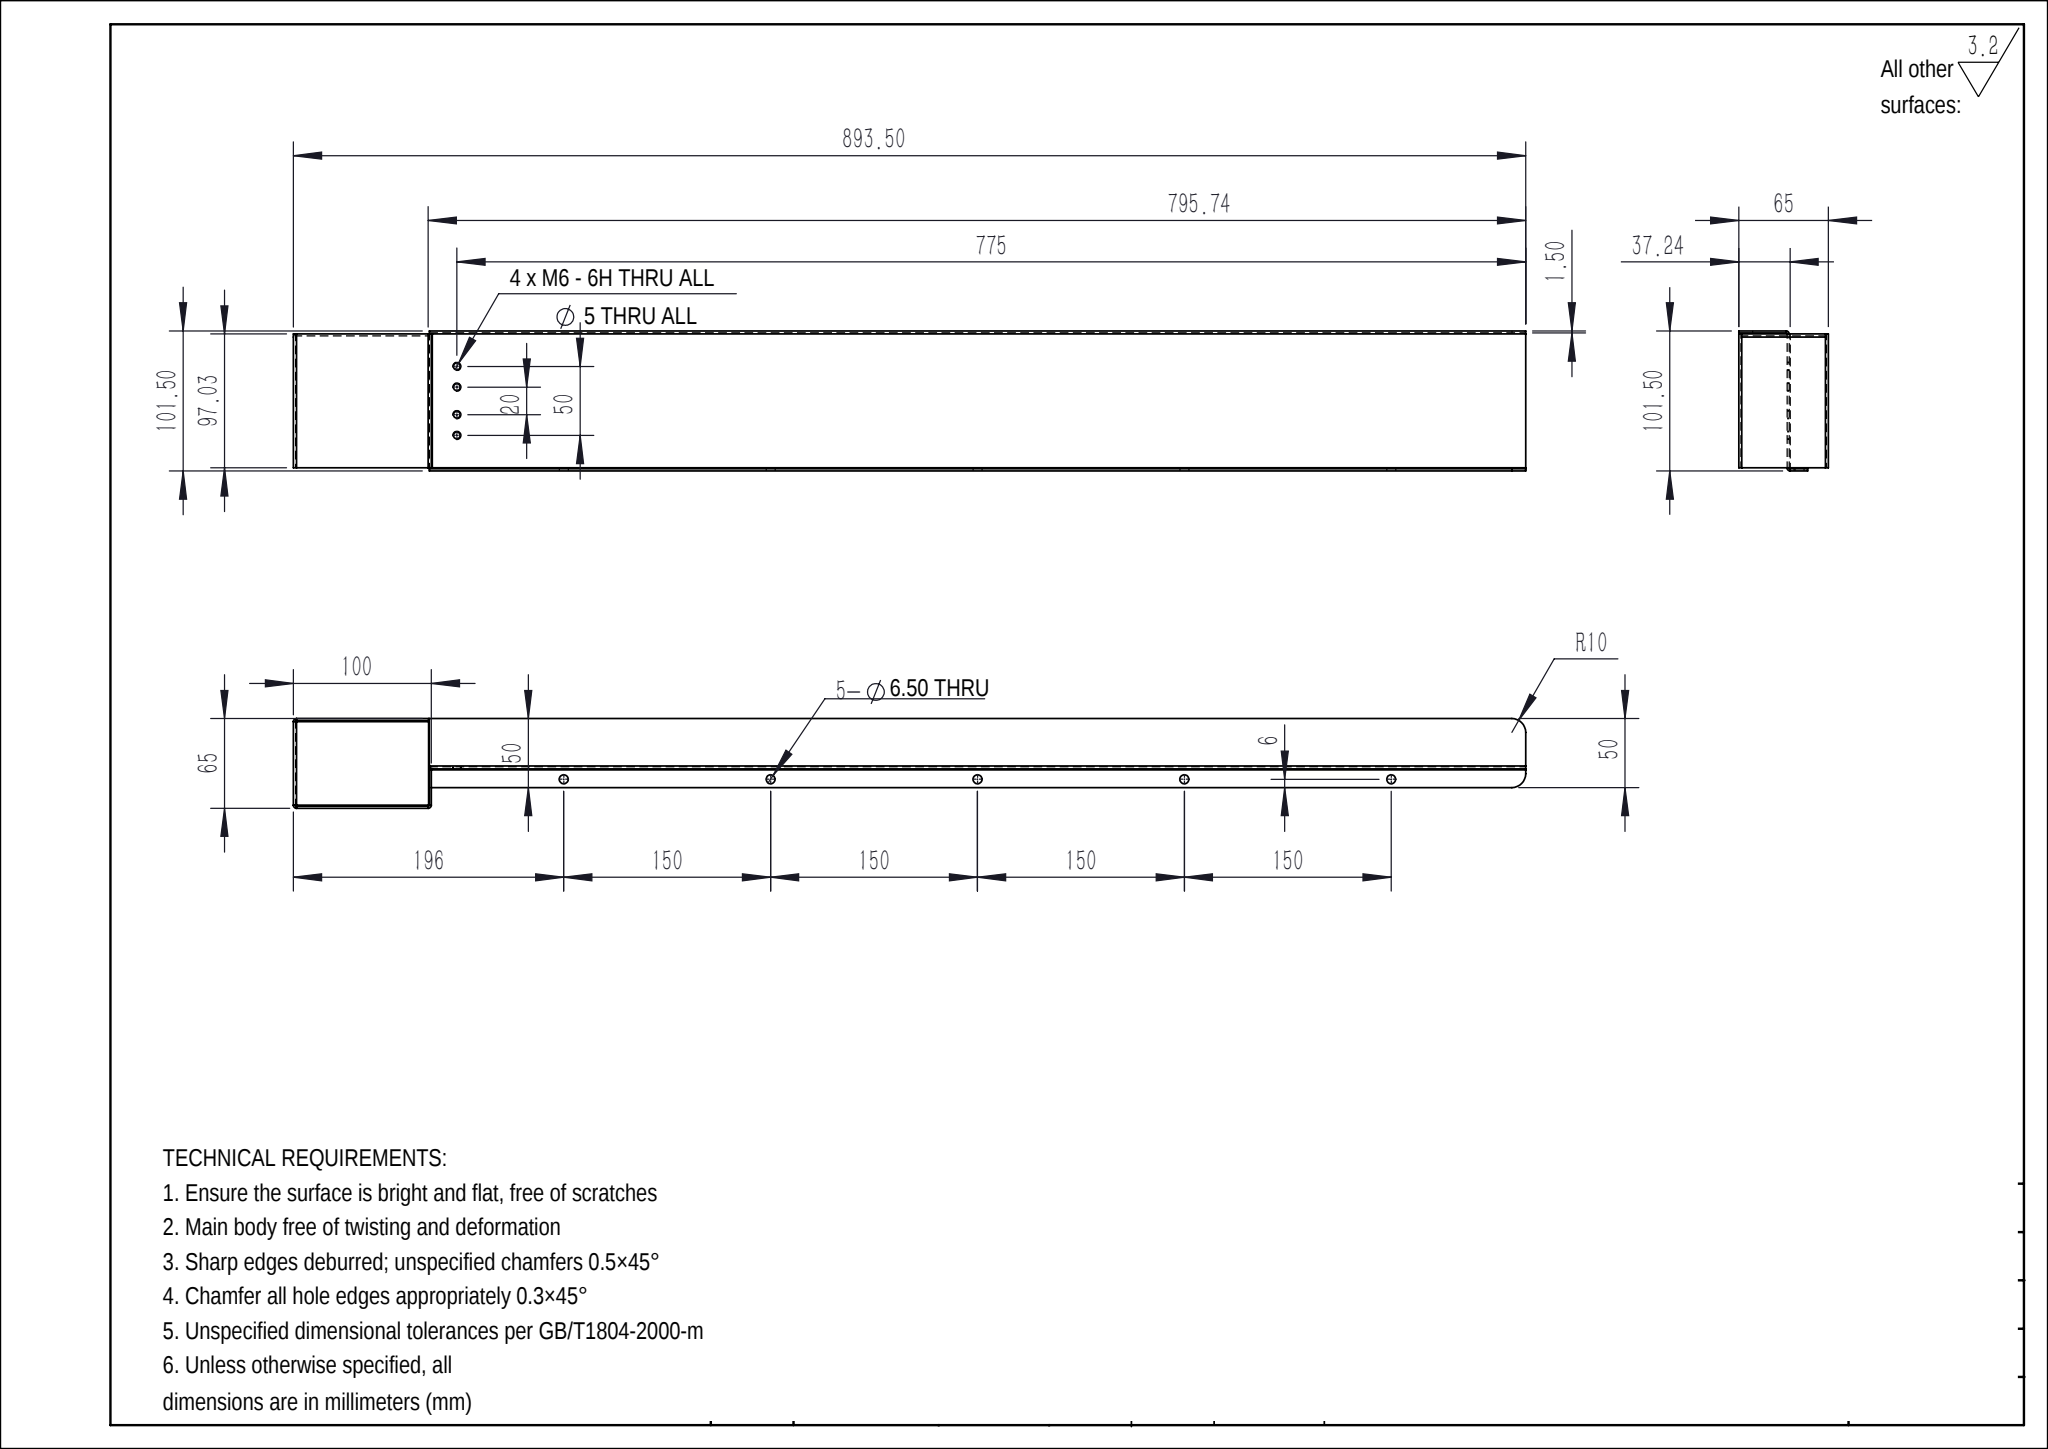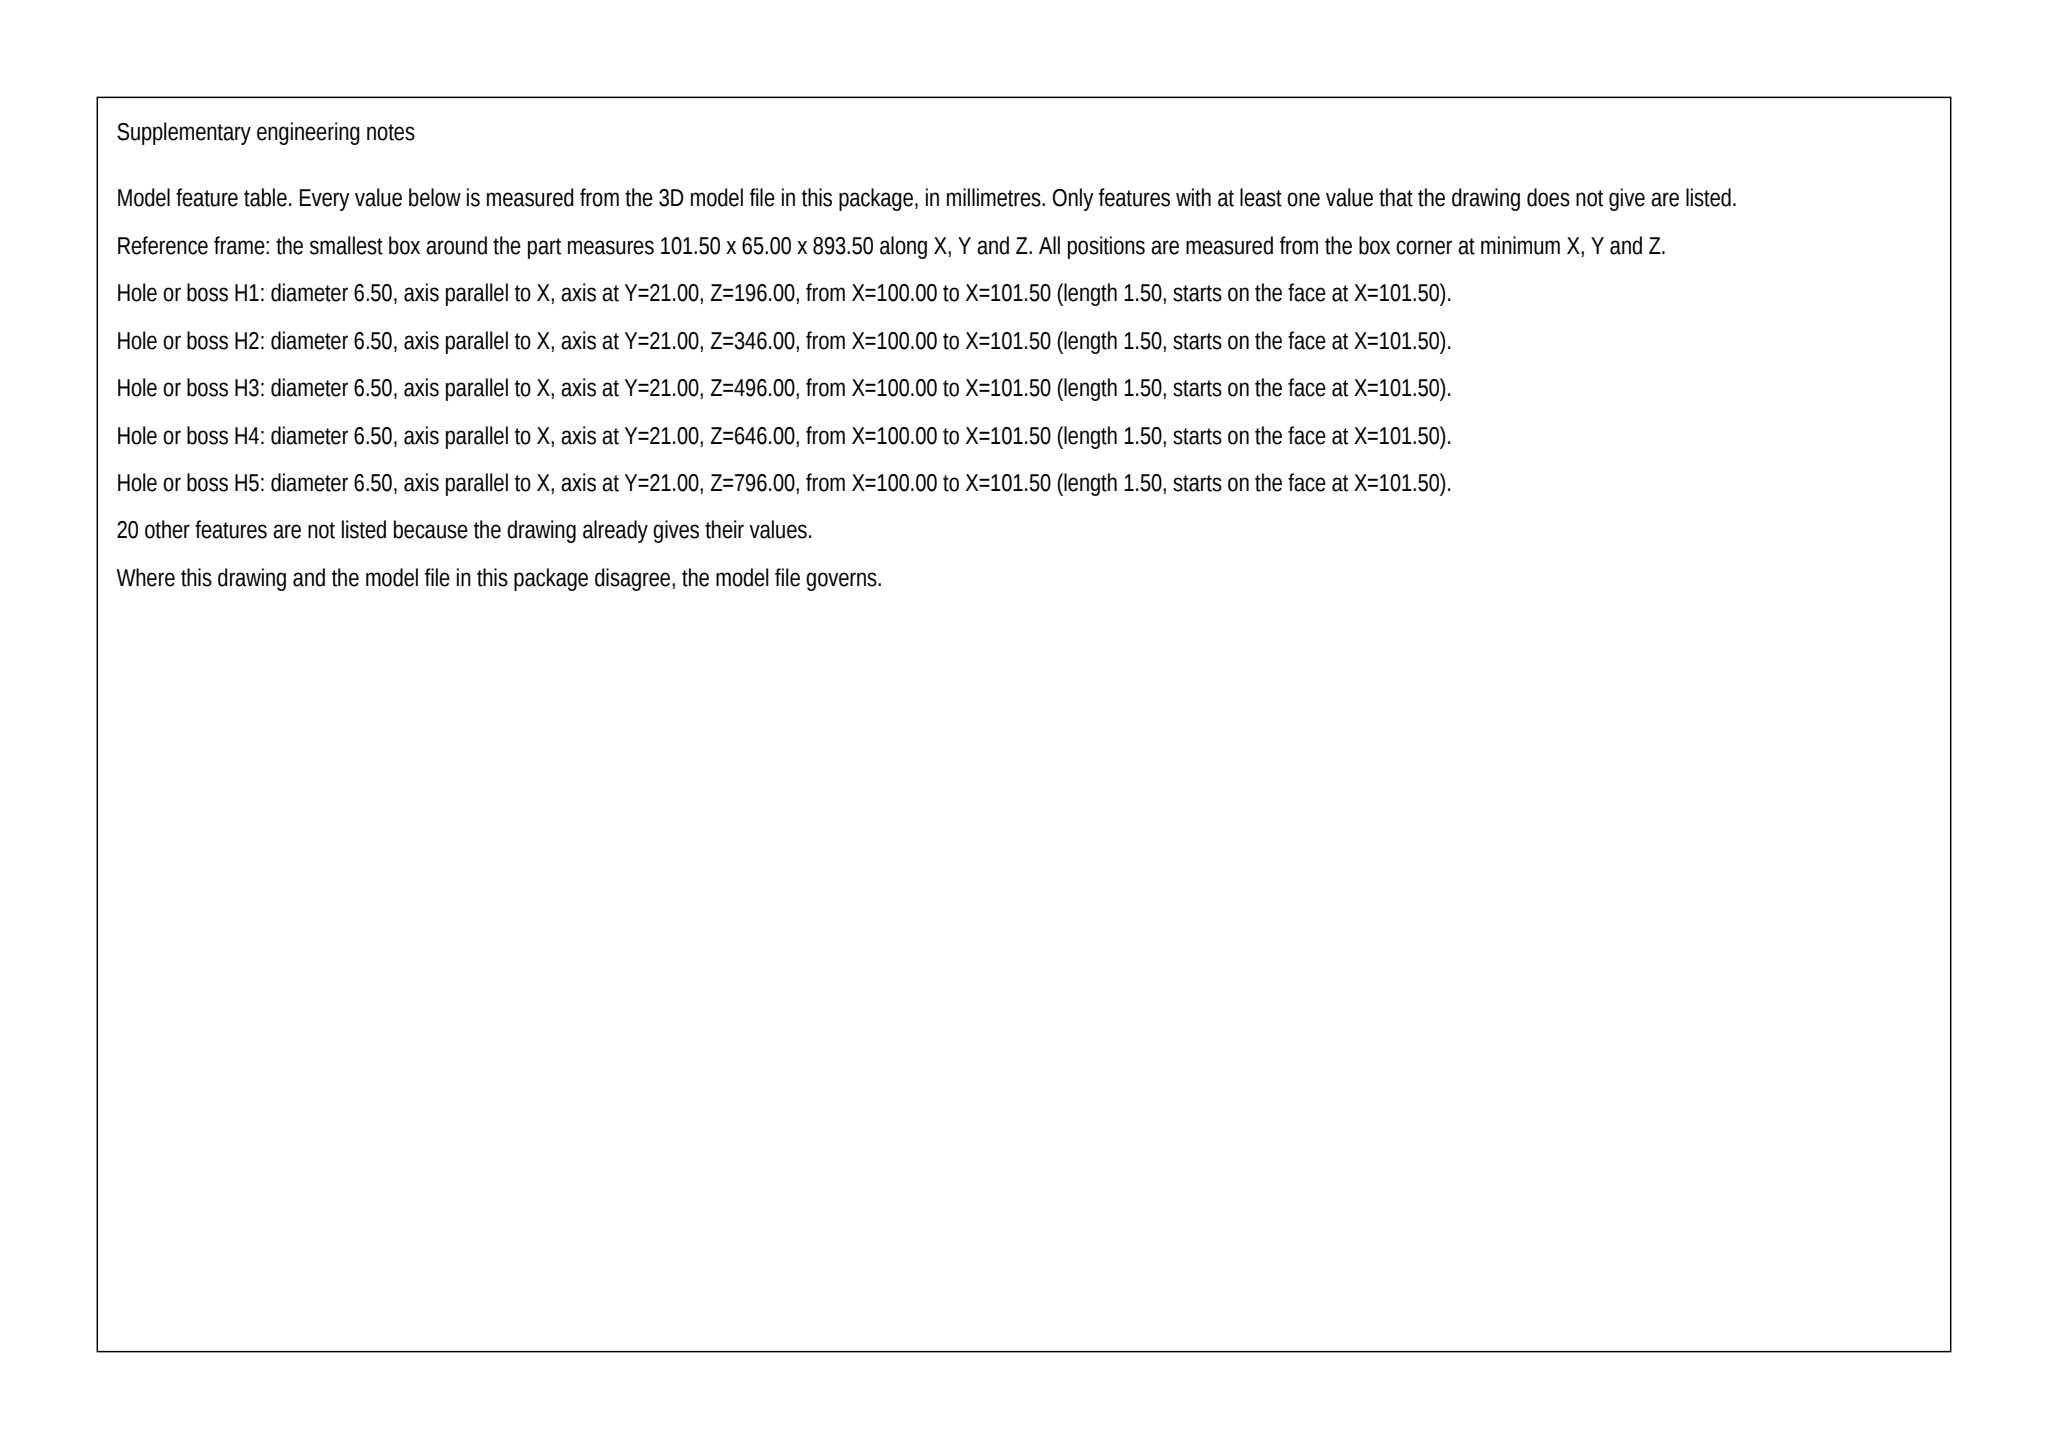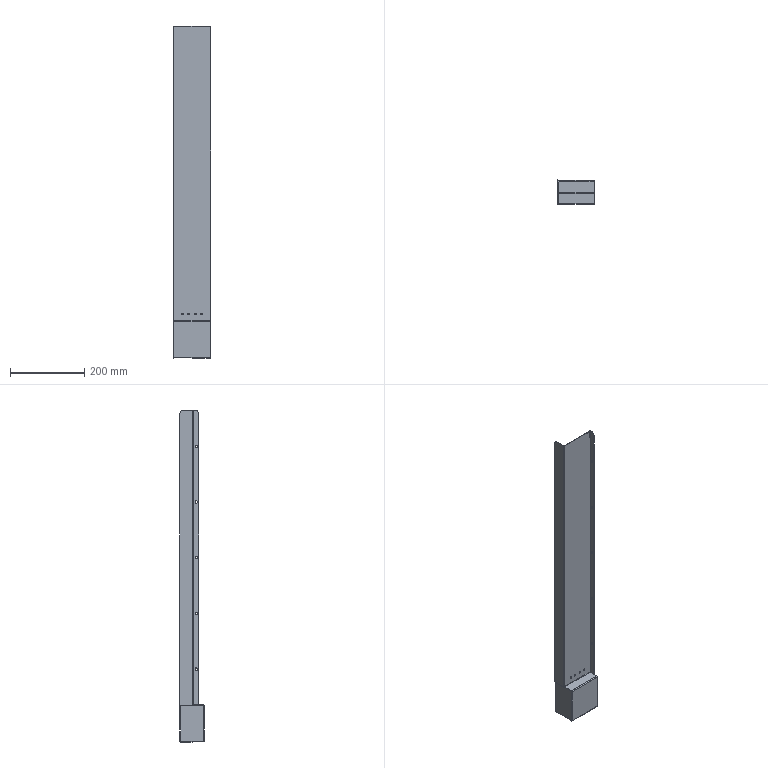Part | SolidWorks | mm | 1 solid | 86 faces | box 101.5 x 65 x 893.5 mm | volume 227024 mm3 | plane 52 | cylinder 34 | commonest cylinder face diameters 6.5 x10 5 x8 4.473 x7 1.473 x7 20 x2
Drawing notes:
4 x M6 HOLE GRP CL 118.50 FROM LH END (893.50 DATUM) | from the solid: Ø5 cylinders, axis y, at z=118.5; bbox z=893.5, LH end z=0
4 x M6 CL SPACING 15, 20, 15 (50 OVERALL) ON 101.50 FACE | from the solid: Ø5/M6 holes at x=25.75, 40.75, 60.75, 75.75; bbox x=101.5
2-Ø20 THRU, CL 883.50 FROM LH END, AT 25 AND 55 ON 65 FACE | from the solid: Ø20 cylinders, axis x, at y=25 and y=55, z=883.5, length 1.5
CHANNEL 50 HT FLUSH W/ TOP OF 65 END BLOCK; 15 STEP AT BOTTOM | from the solid: y-planes 0,15,65: block y0-65 (65), channel y15-65 (50); Ø6.5 holes at y=21 = 6 up from y=15 channel bottom
LH END CLOSURE FLG: 1.5 THK x 60.53 LG, BENT 90, R0.74 INSIDE | from the solid: z-planes 0 & 1.5 at LH end; bend cyls dia 1.473/4.473 axis Y at x=4.47,z=2.24, length 60.53 (y 2.24-62.76)
LH END FLANGE 1.5 THK x 60.53 LG: BEND LINE 4.47 FROM 101.50 EDGE | from the solid: Cyl axis y at x=4.47, z=2.24, len 60.53, R0.7365 inner bend; plane x=3.74 flange inner face
END VIEW: SECTION 101.50 x 65 OA; 65 = FULL WIDTH, 37.24 REF ONLY | from the solid: bbox_xyz 101.5 x 65.0; planes y=0 and y=65, x=0 and x=101.5 bound section (37.24+65=102.24 does not close)
2-Ø20 THRU ONE 1.5 WALL ONLY, 25 & 55 FROM 65 EDGE, 10 FROM RH END | from the solid: Cyl Ø20 axis x at y=25.0 and y=55.0, z=883.5, length 1.5, count 1 (one wall); 893.5-883.5=10
CHANNEL BOTTOM RETURN LIP: 1.5 THK, FULL 795 LG; LIP FACES AT 28.50 AND 30.00 FROM THE 65 DATUM EDGE (Y0); BEND CL 27.76 (RH WALL) AND 30.74 (LH WALL), R0.74 INSIDE. 37.24 IN END VIEW IS REF ONLY. | from the solid: axis_planes y=28.5 and y=30.0 (1.5 thk lip); z-axis bend cylinders dia 1.473/4.473 at [99.26,27.76] and [2.24,30.74], length 795 (R0.74 inside / R2.24 outside)
CHANNEL BOTTOM RETURN LIP (BOTH 1.5 WALLS): 1.5 THK, LIP INNER FACE 28.50 AND OUTER FACE 30.00 FROM 65 DATUM EDGE (Y0); LIP RUNS FROM 98.50 TO 893.50 FROM LH END (795.00 LG) | from the solid: axis_planes y=28.5 and y=30.0; z-axis cylinders dia1.473/4.473 at [2.24,30.74] and [99.26,27.76], length 795.0 between z-planes 98.5 and 893.5
LIP BEND CL 27.76 FROM 65 DATUM EDGE ON 99.26 WALL AND 30.74 ON 2.24 WALL; R0.74 INSIDE ALL BENDS | from the solid: z-axis cylinders dia 1.473 (R0.7365) at [2.24,30.74] and [99.26,27.76]; x-axis dia 1.473 at y=2.24/27.76/62.76
4X M6-6H (Ø5 DRILL) ON 101.50 FACE: HOLE CLS 25.75, 40.75, 60.75, 75.75 FROM X0 EDGE OF 101.50 FACE, ALL 118.50 FROM LH END | from the solid: y-axis cylinders dia 5.0 at [25.75,118.5], [40.75,118.5], [60.75,118.5], [75.75,118.5], length 1.5